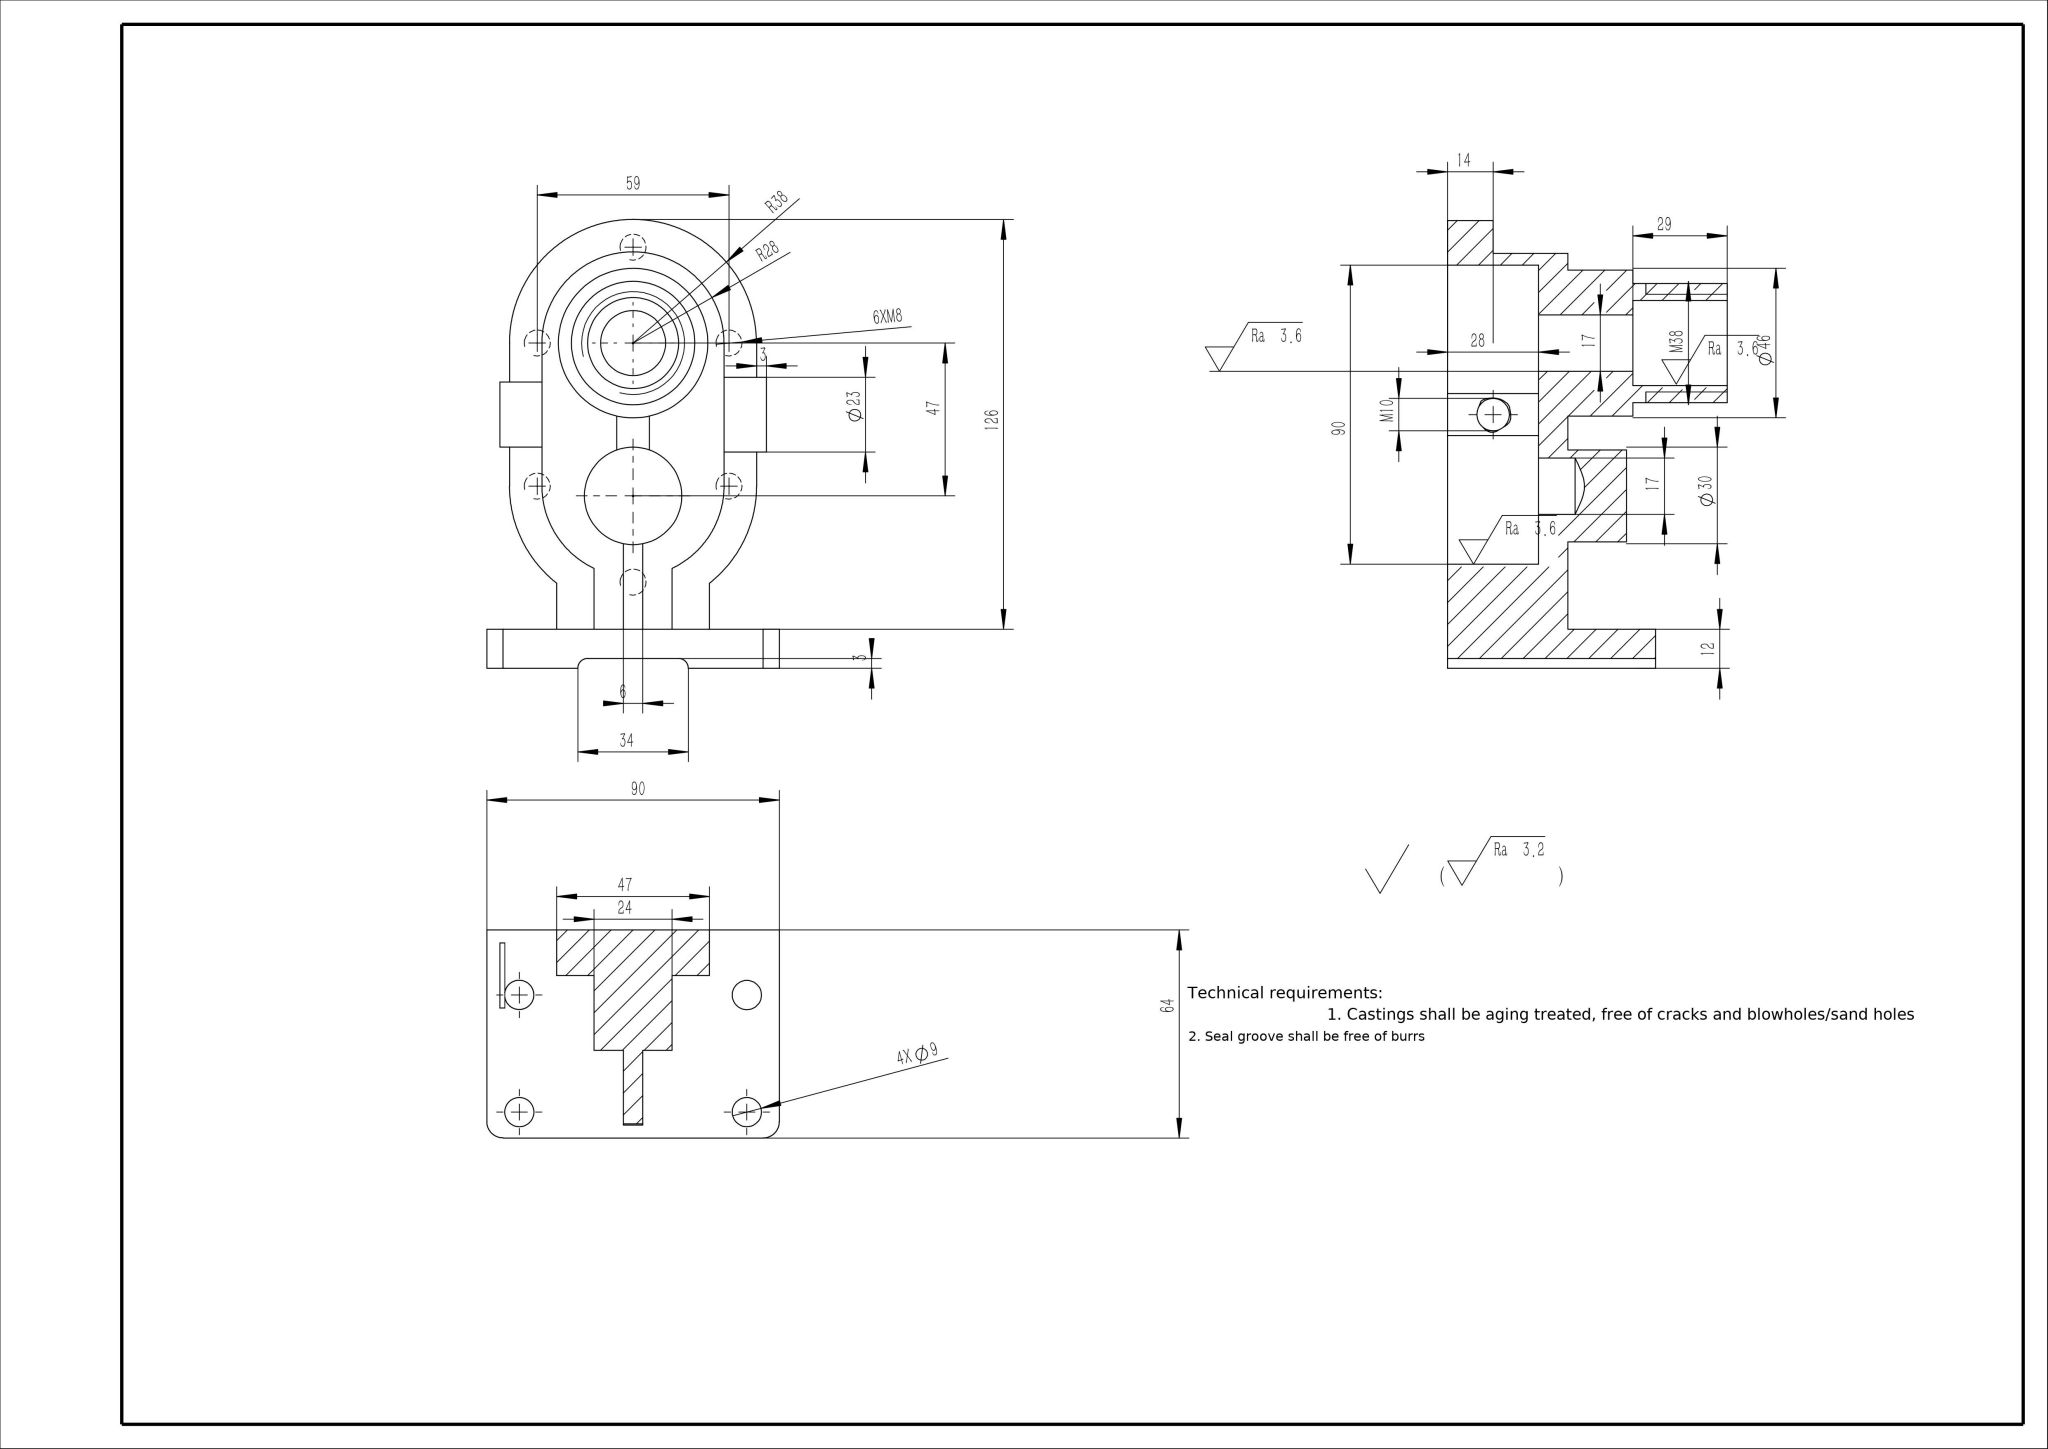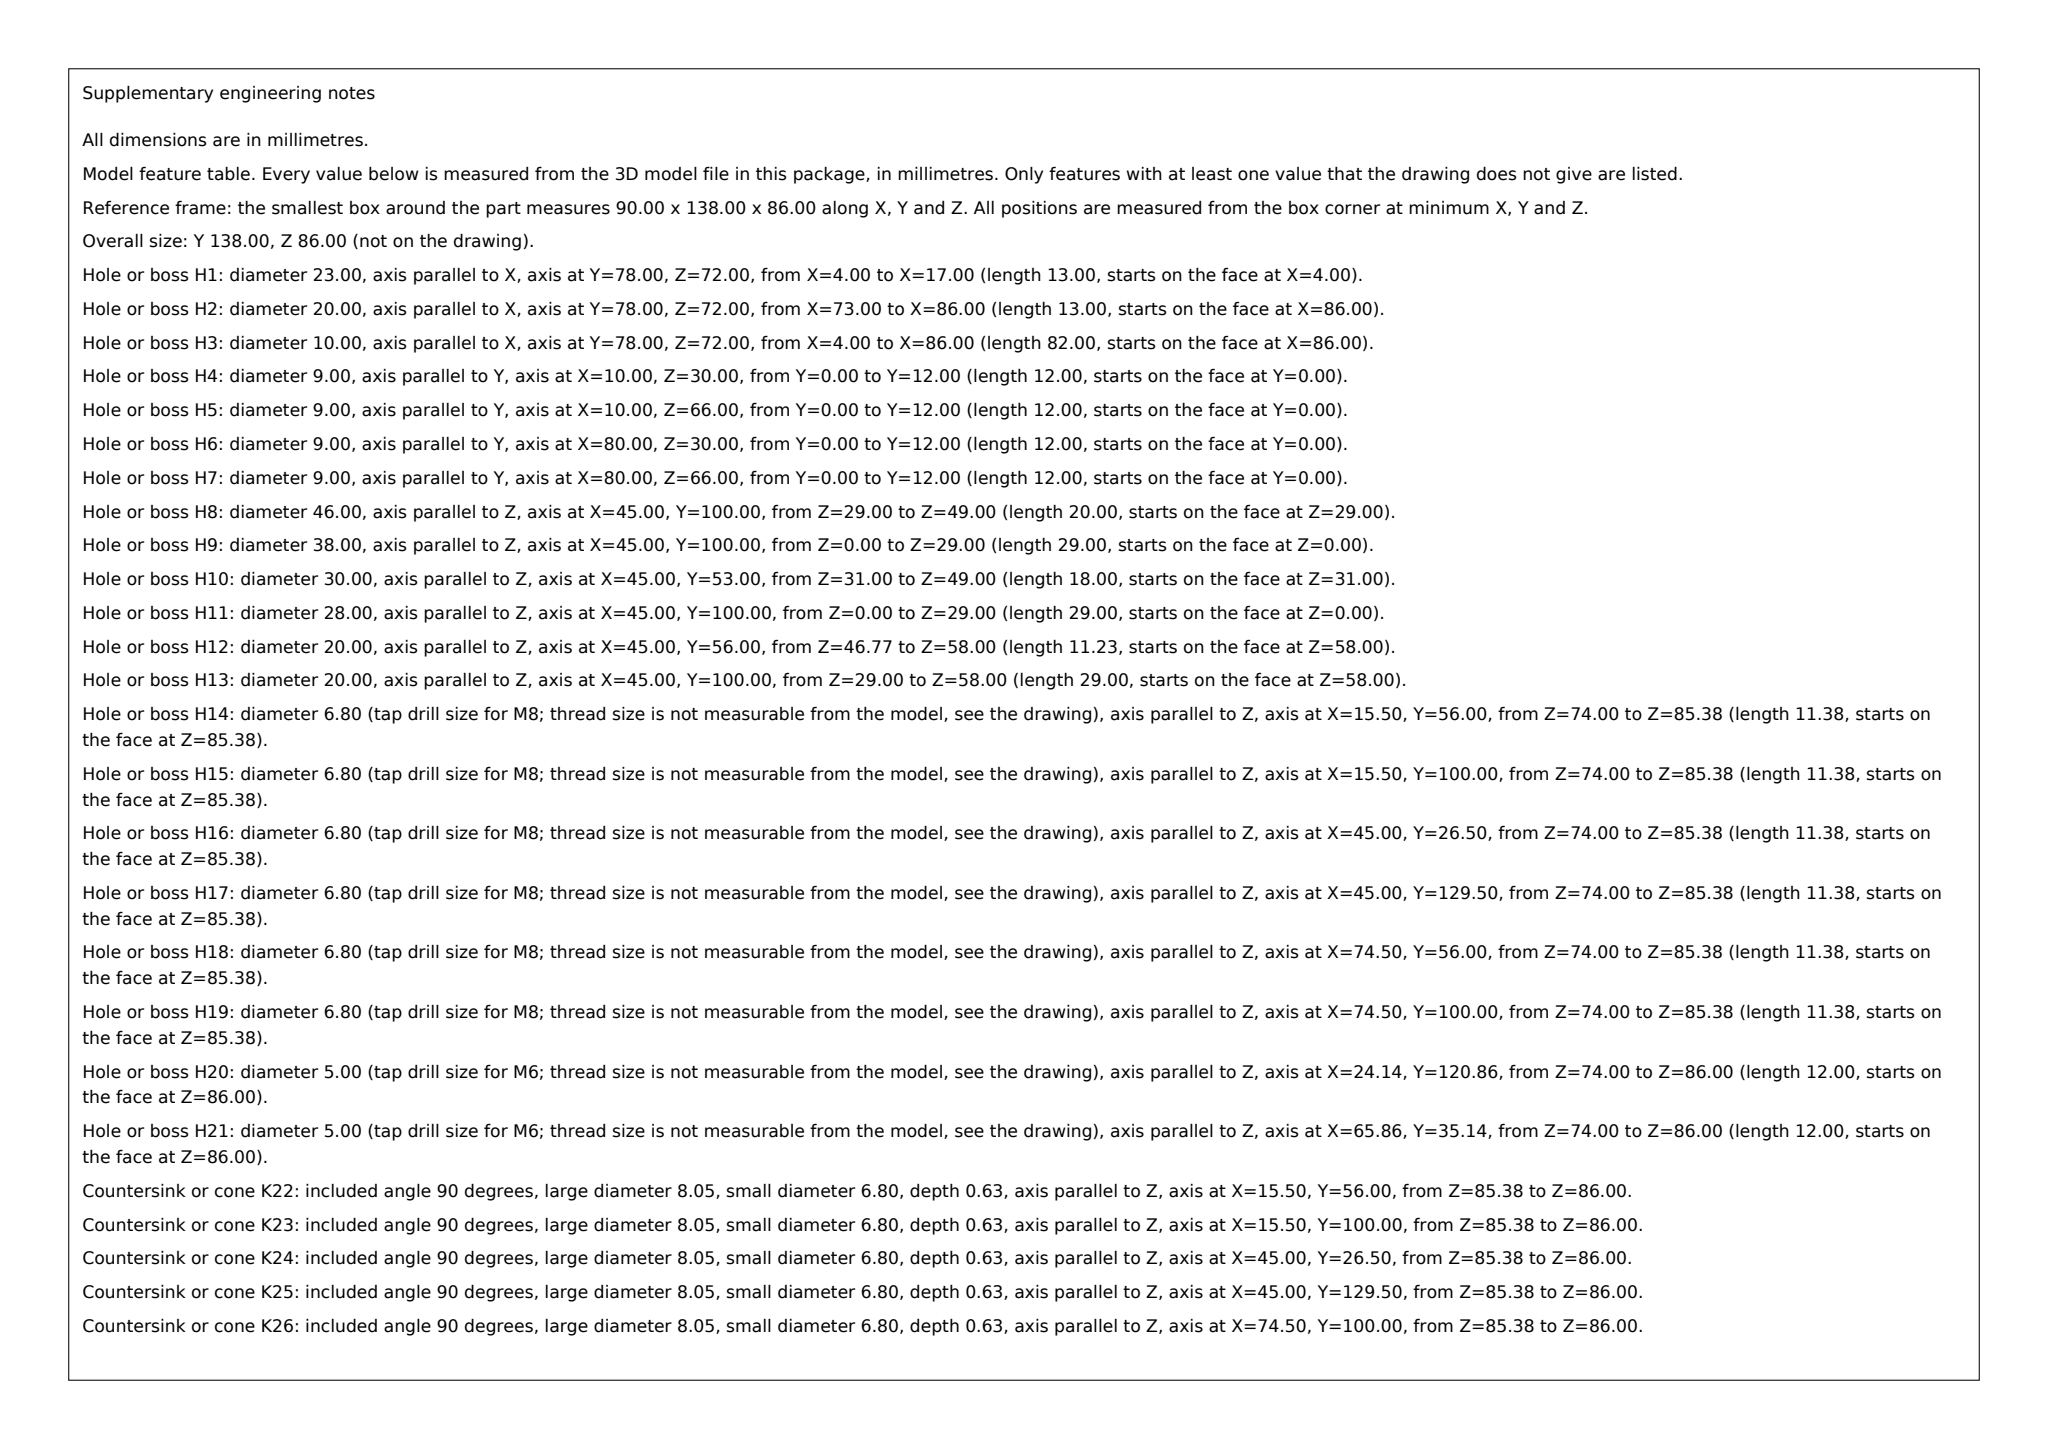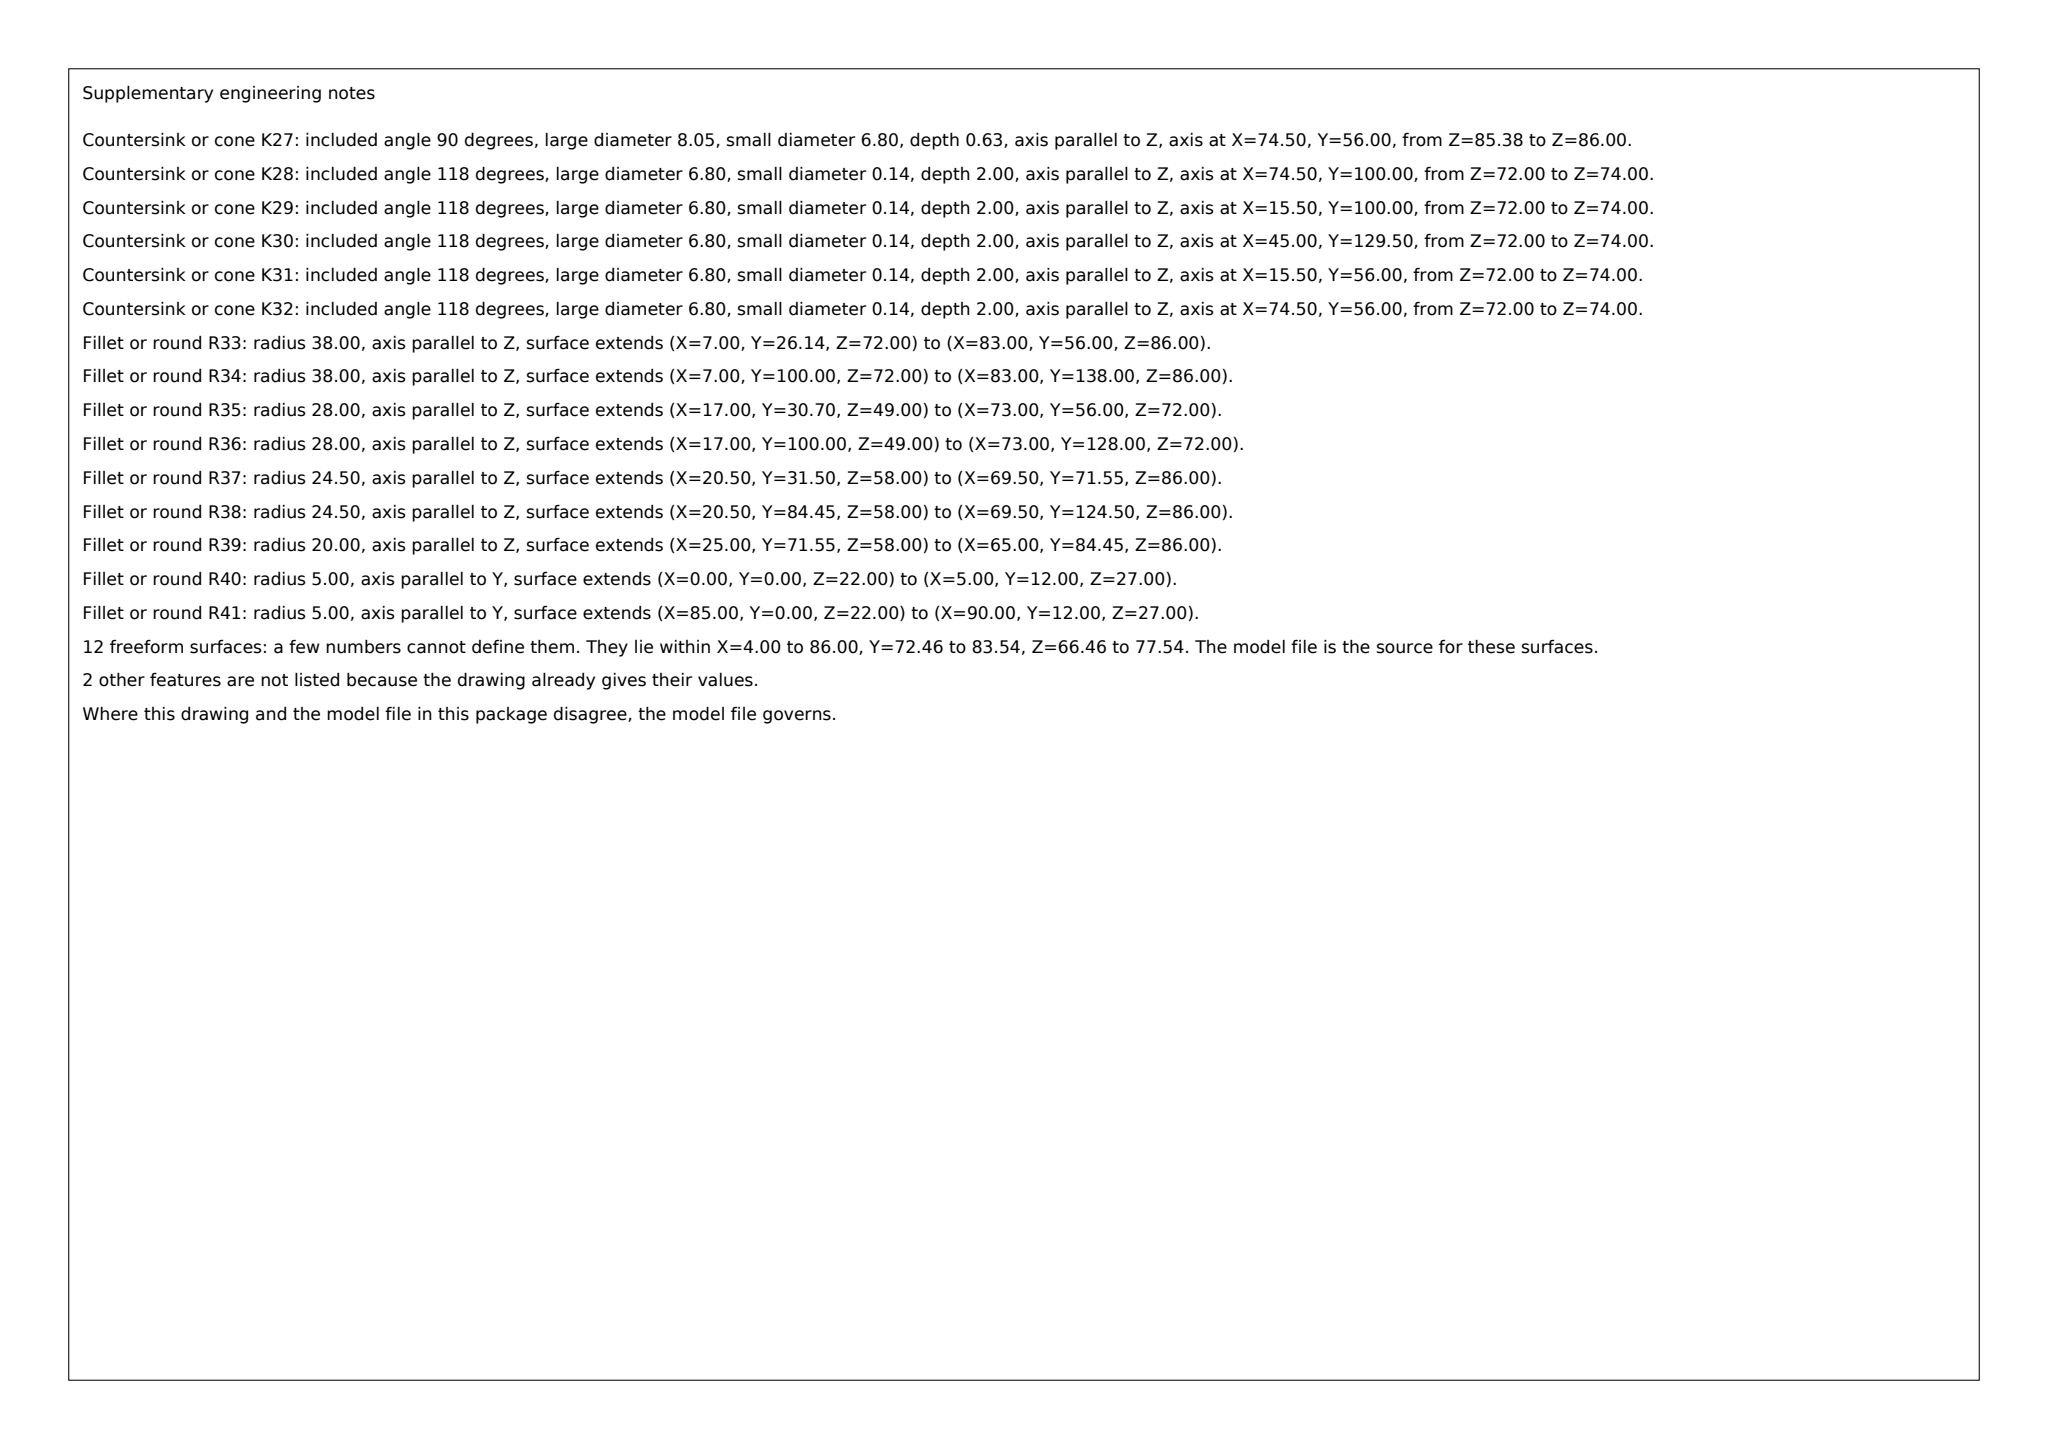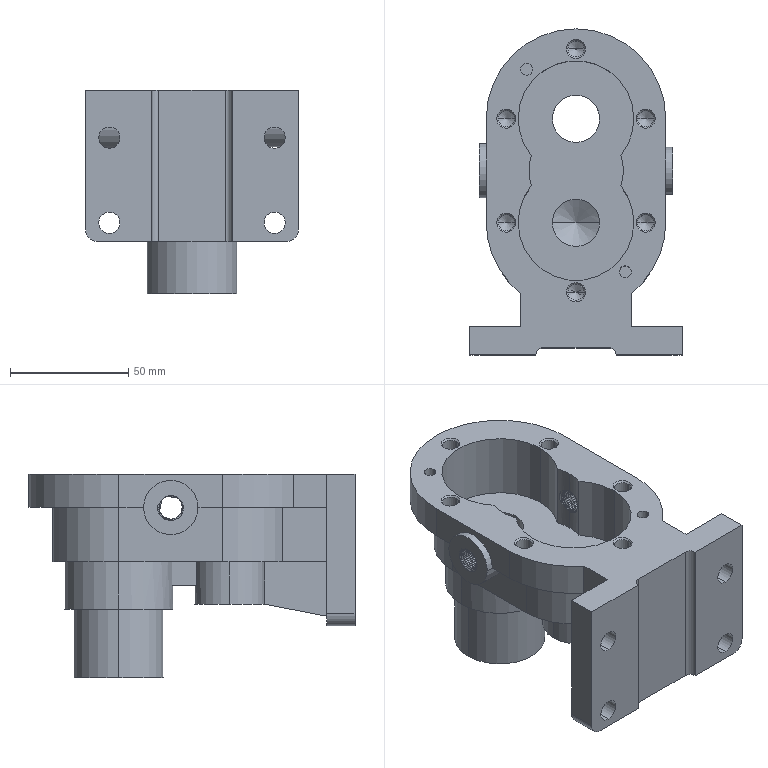Part | SolidWorks | mm | 1 solid | 225 faces | box 90 x 138 x 86 mm | volume 242506 mm3 | cylinder 151 | plane 36 | cone 26 | spline 12 | commonest cylinder face diameters 10 x93 6.8 x12 9 x8 20 x6 49 x6 5 x4 30 x3 40 x3